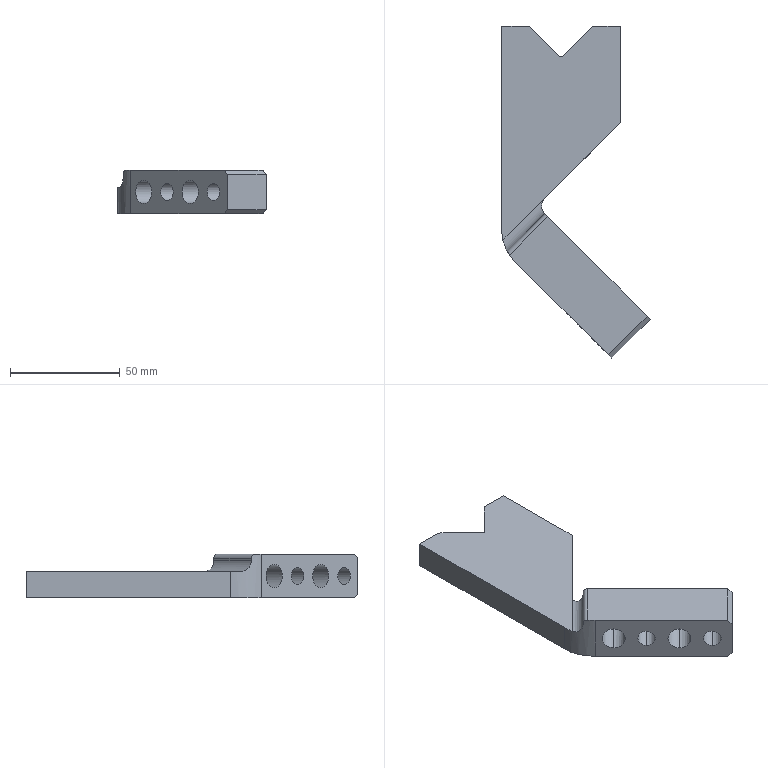CAM job | Mastercam | mm | 9 operations | part box 67.66 x 151.38 x 20
1. Drill/Counterbore | 2 - D6-A90.0点孔倒角刀
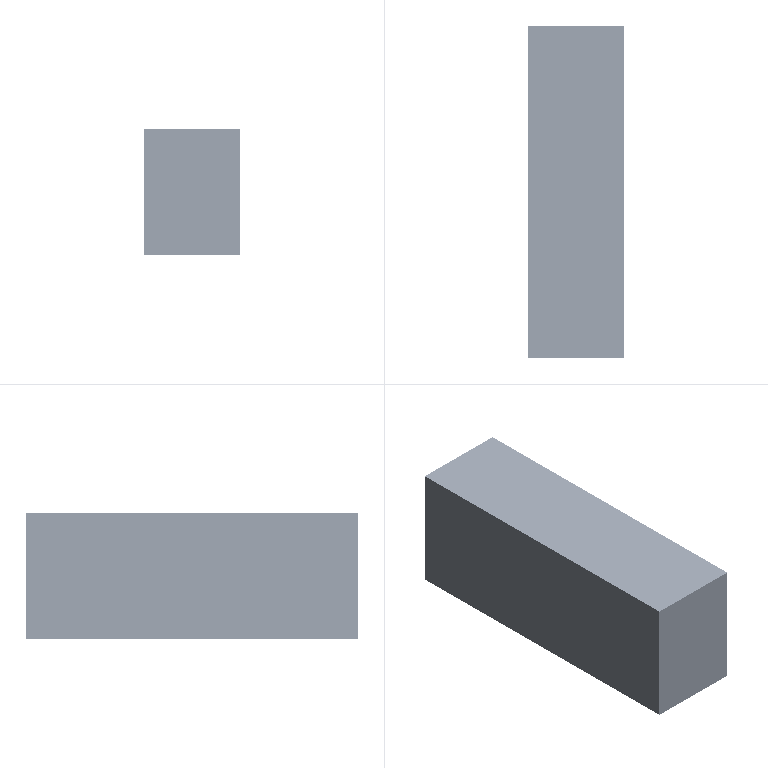2. Peck Drill | 19 - 7.9 钻头
3. Peck Drill | 20 - 10.5 钻头
4. Model Chamfer | 15 - D12-A45刀片倒角刀
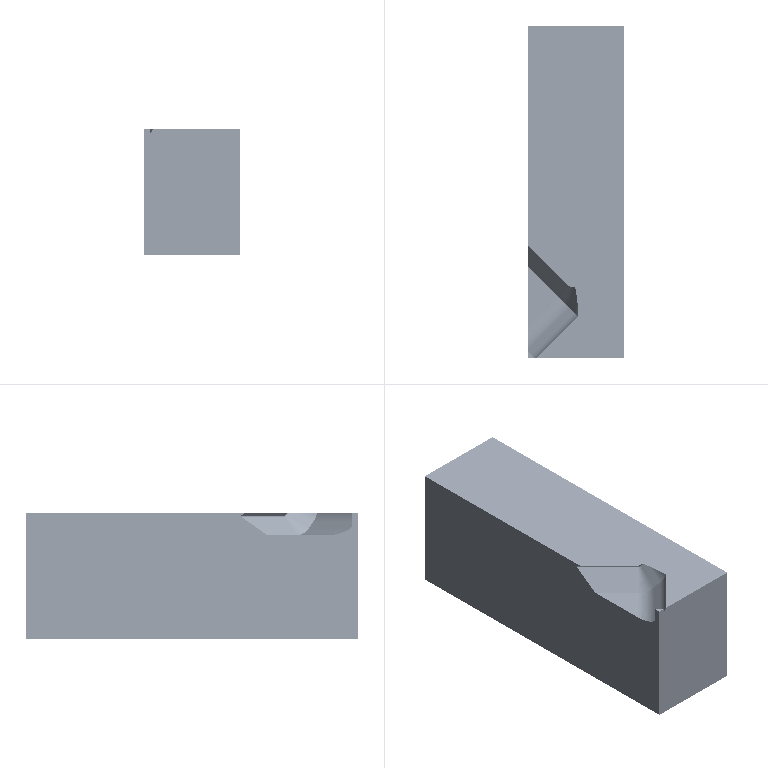5. Advanced Drill | 14 - 8 铰刀
6. Drill/Counterbore | 2 - D6-A90.0点孔倒角刀
7. Peck Drill | 20 - 5 钻头
8. Contour (2D chamfer) | 15 - D12-A45刀片倒角刀
9. Tap | 23 - M6-1.0 右牙